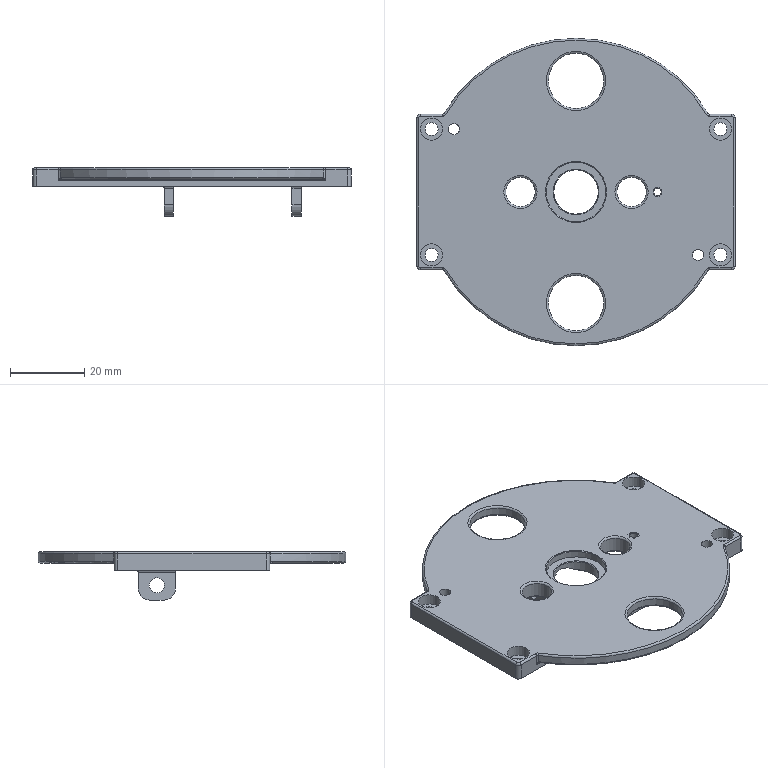Component | NX | DJZ_06_BRACKET2 | 1 solid | 103 faces | volume 21179 mm3 | cylinder 48 | plane 24 | torus 16 | spline 10 | cone 5 | commonest cylinder face diameters 1 x18 6 x8 3.5 x4 2 x4 4.05 x2 3 x2 83 x2 8 x2